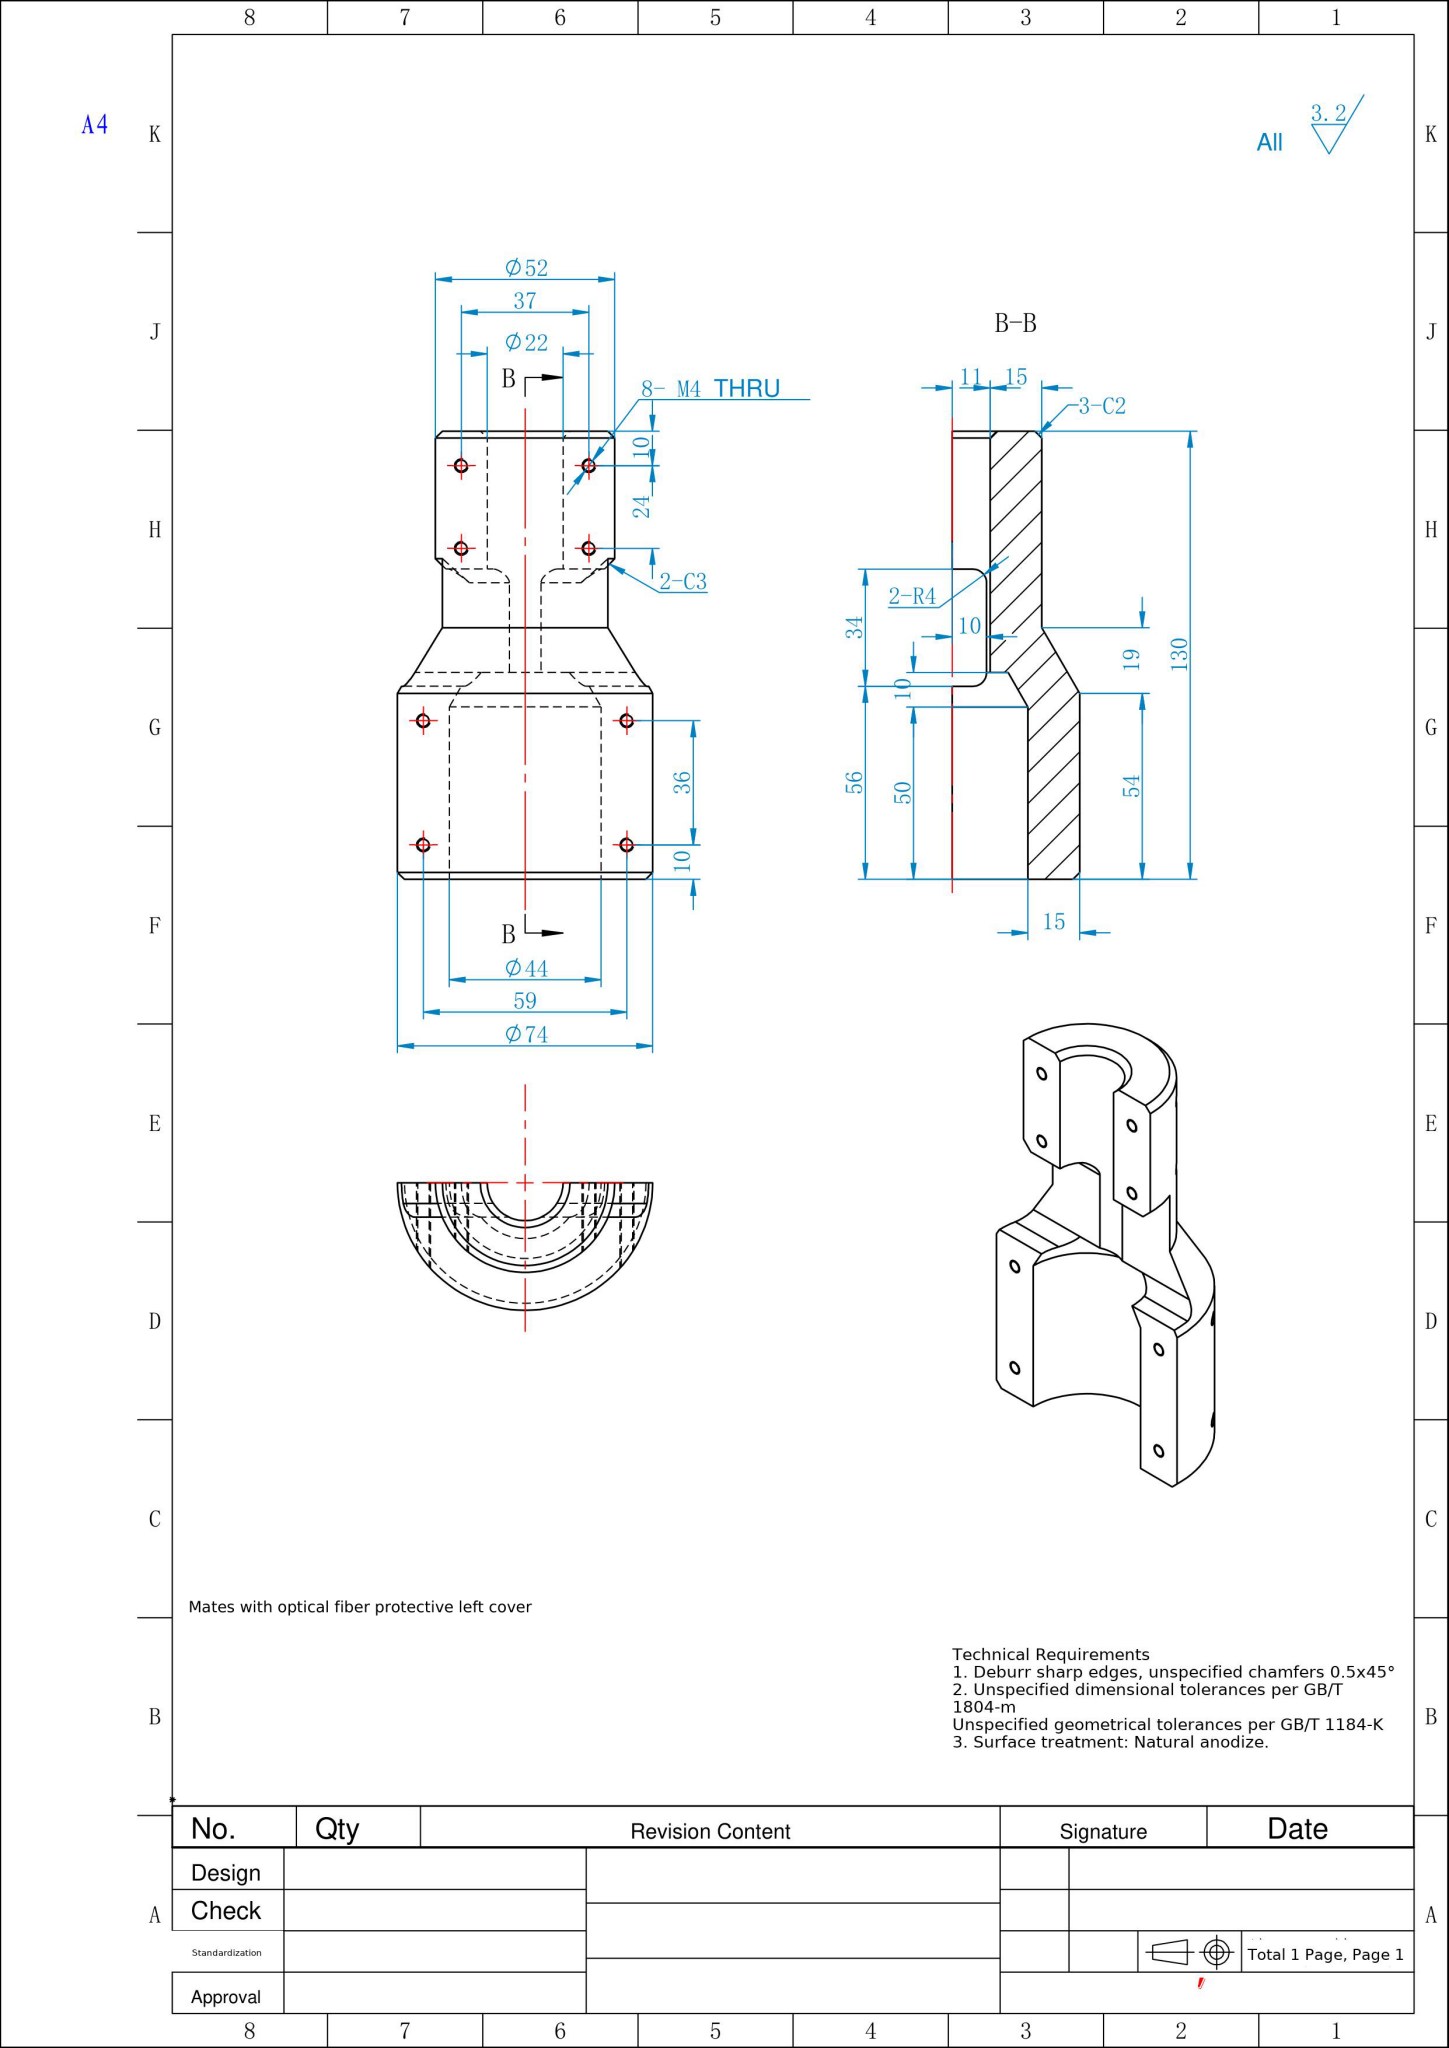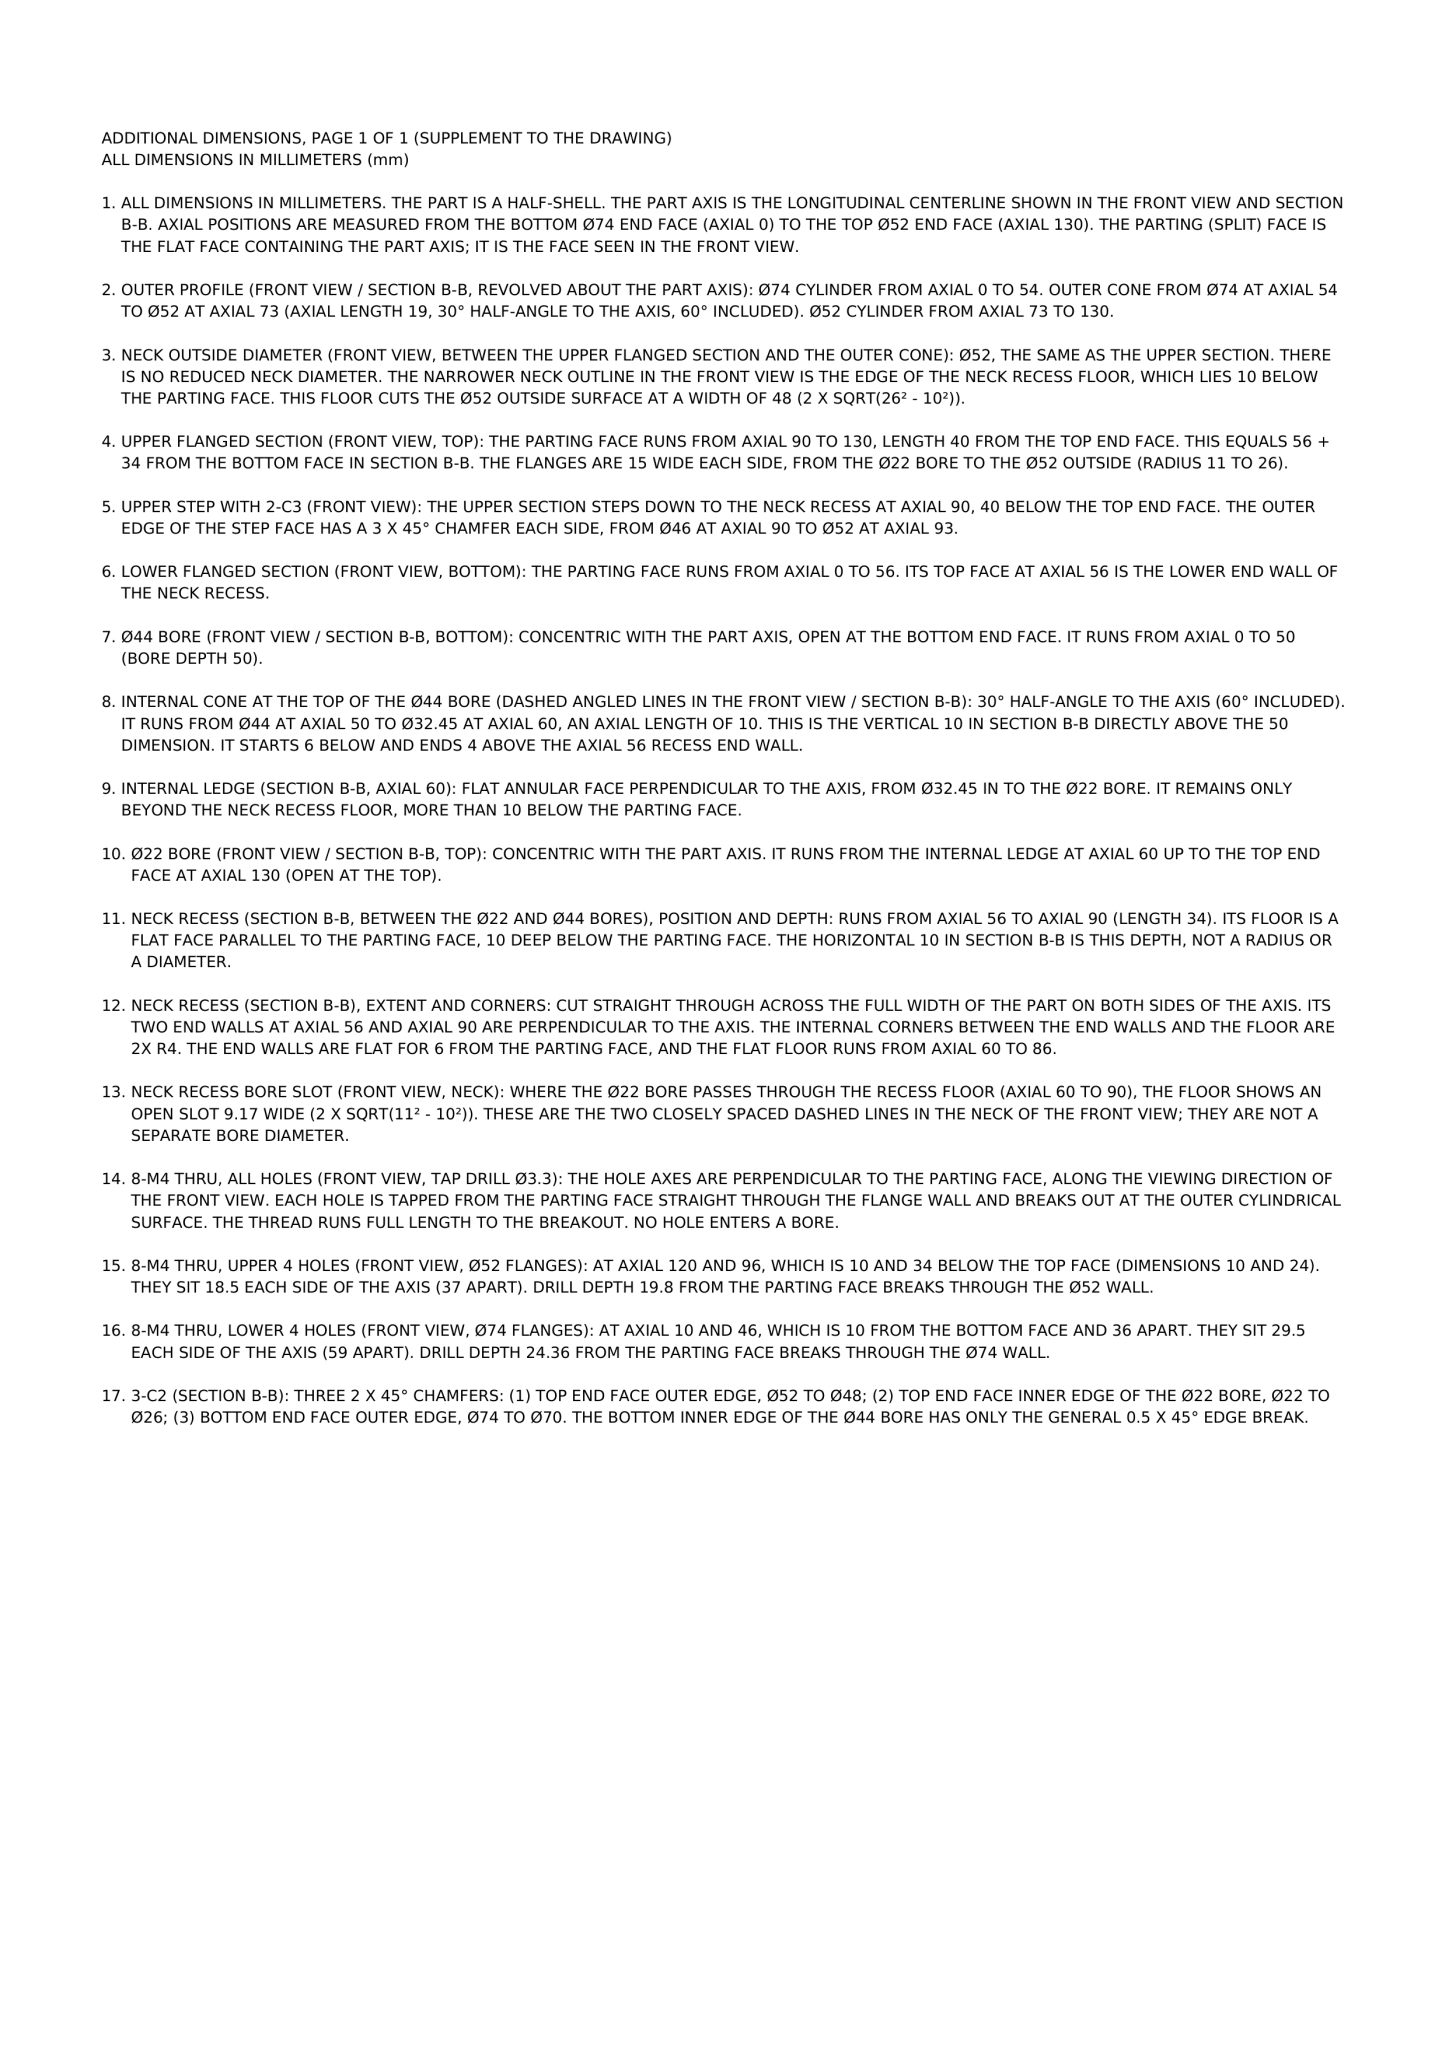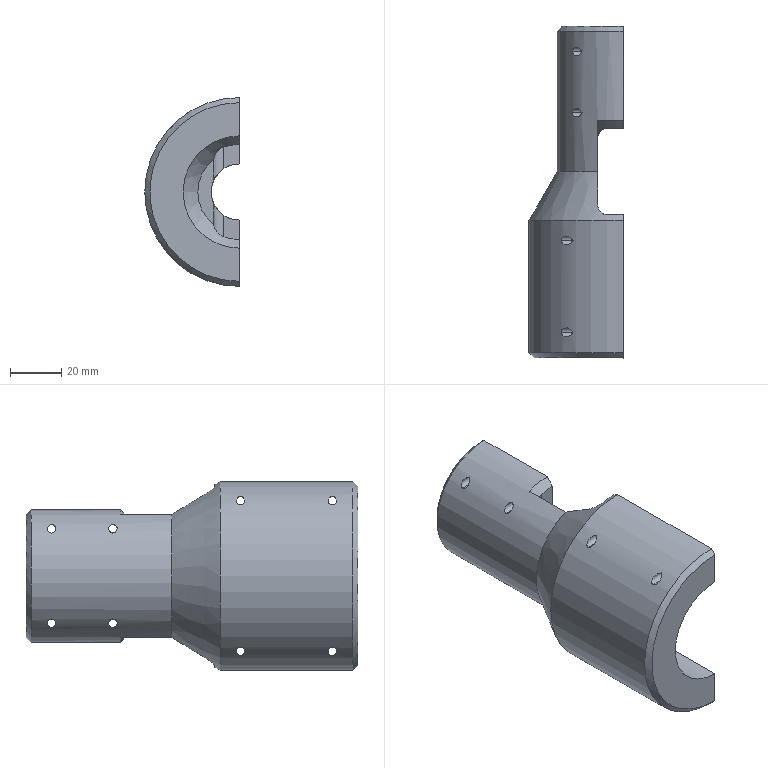Part | NX | mm | 1 solid | 44 faces | box 37 x 130 x 74 mm | volume 135607 mm3 | cylinder 24 | plane 13 | cone 7 | commonest cylinder face diameters 3.3 x16 8 x4 52 x1 74 x1 44 x1 22 x1